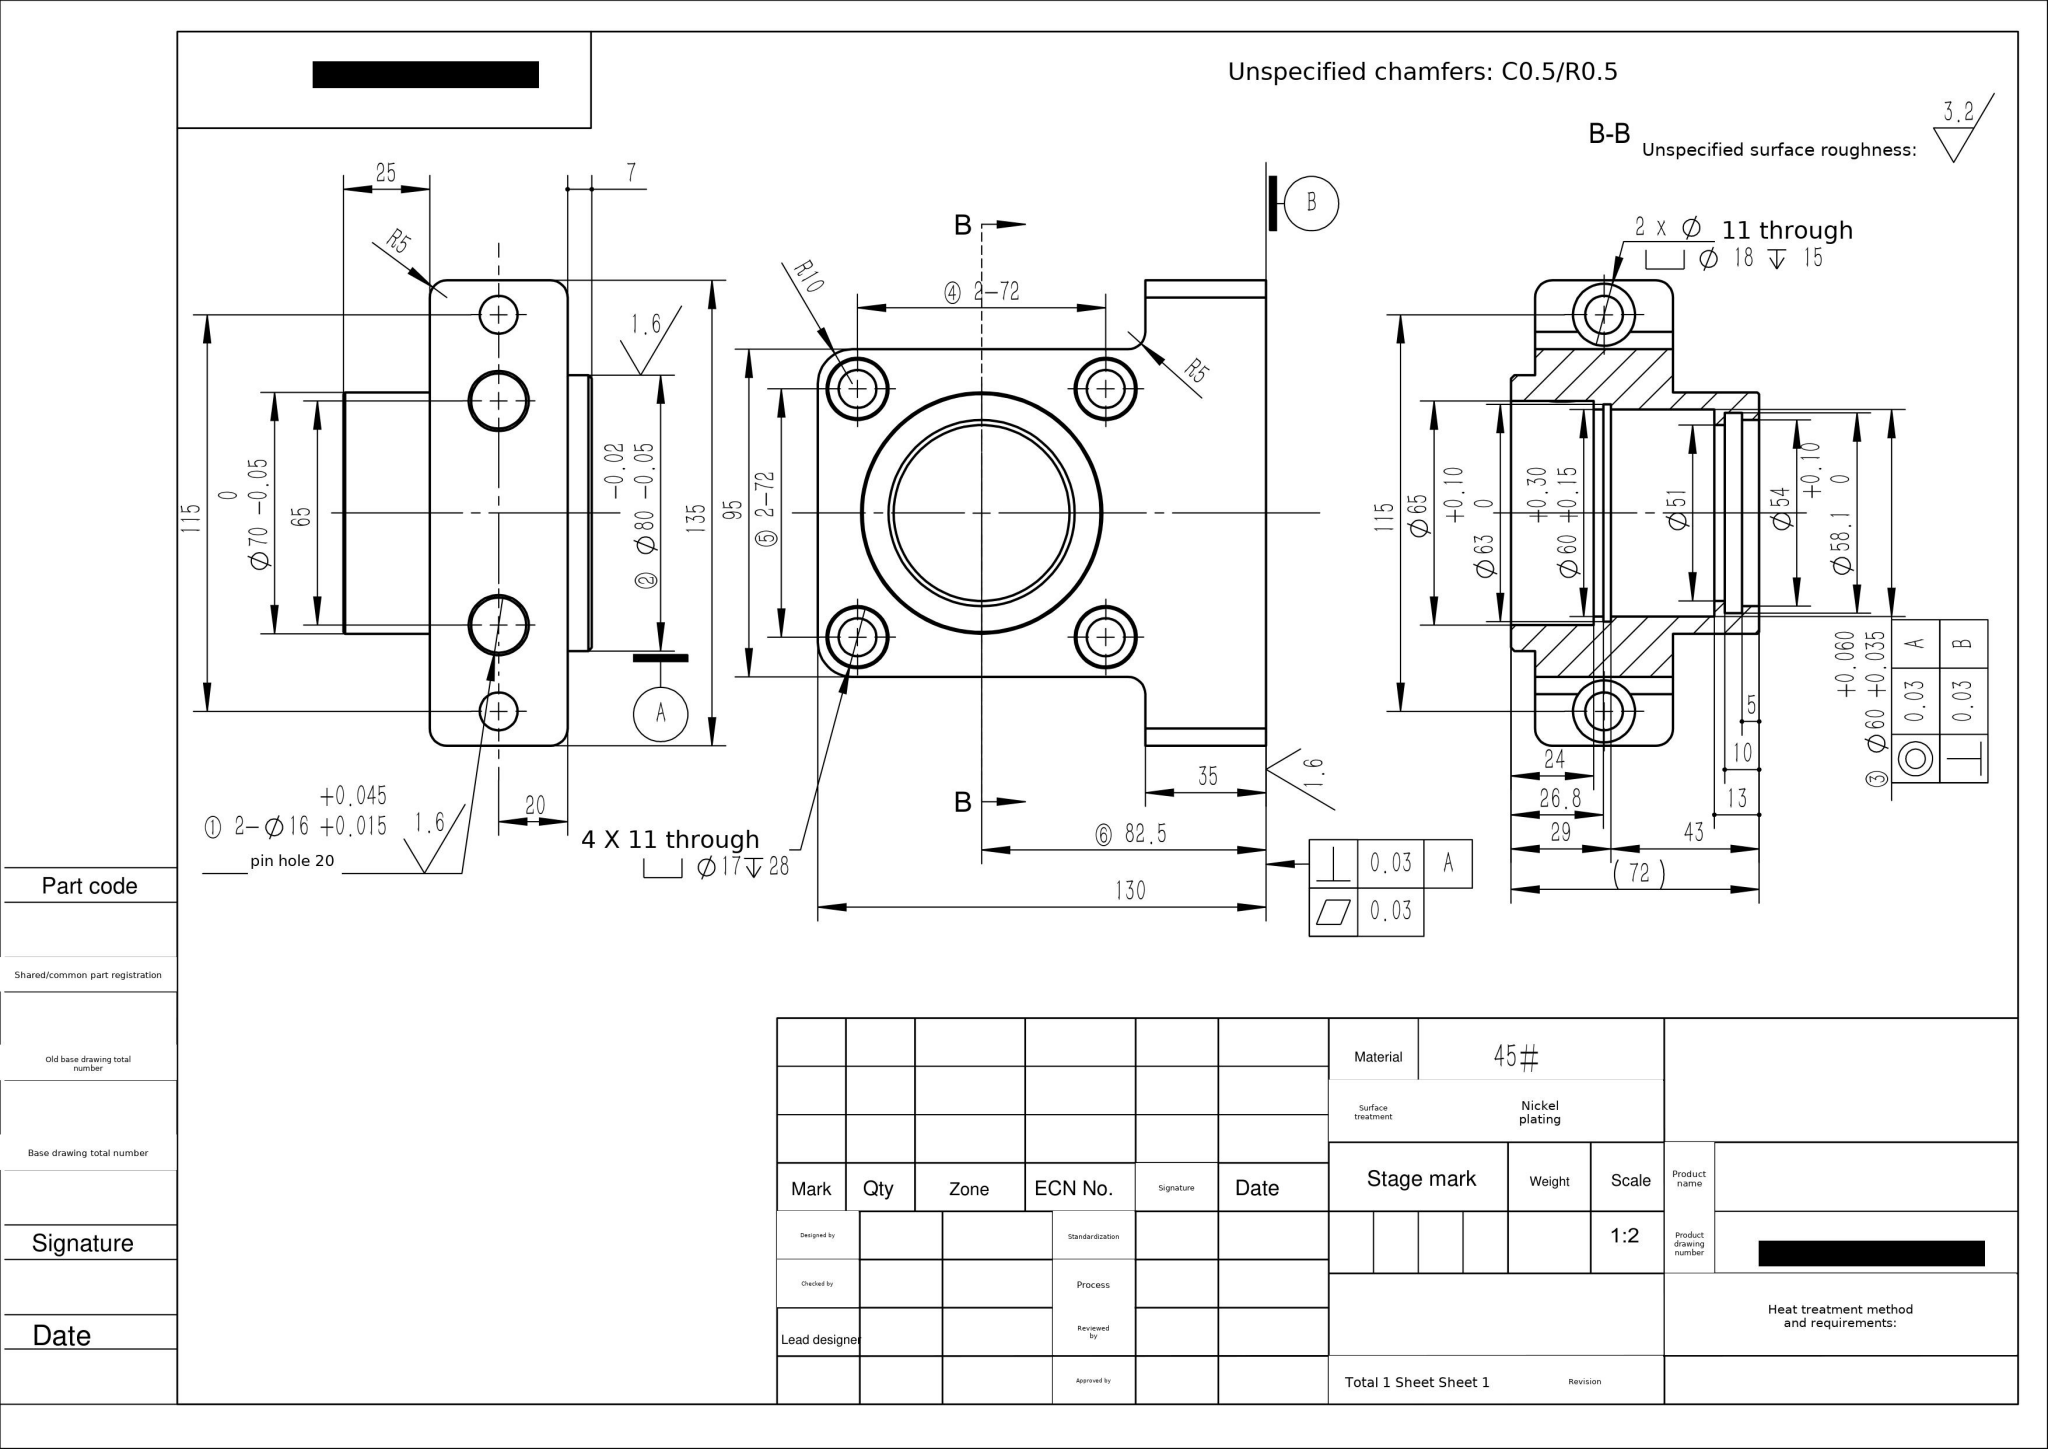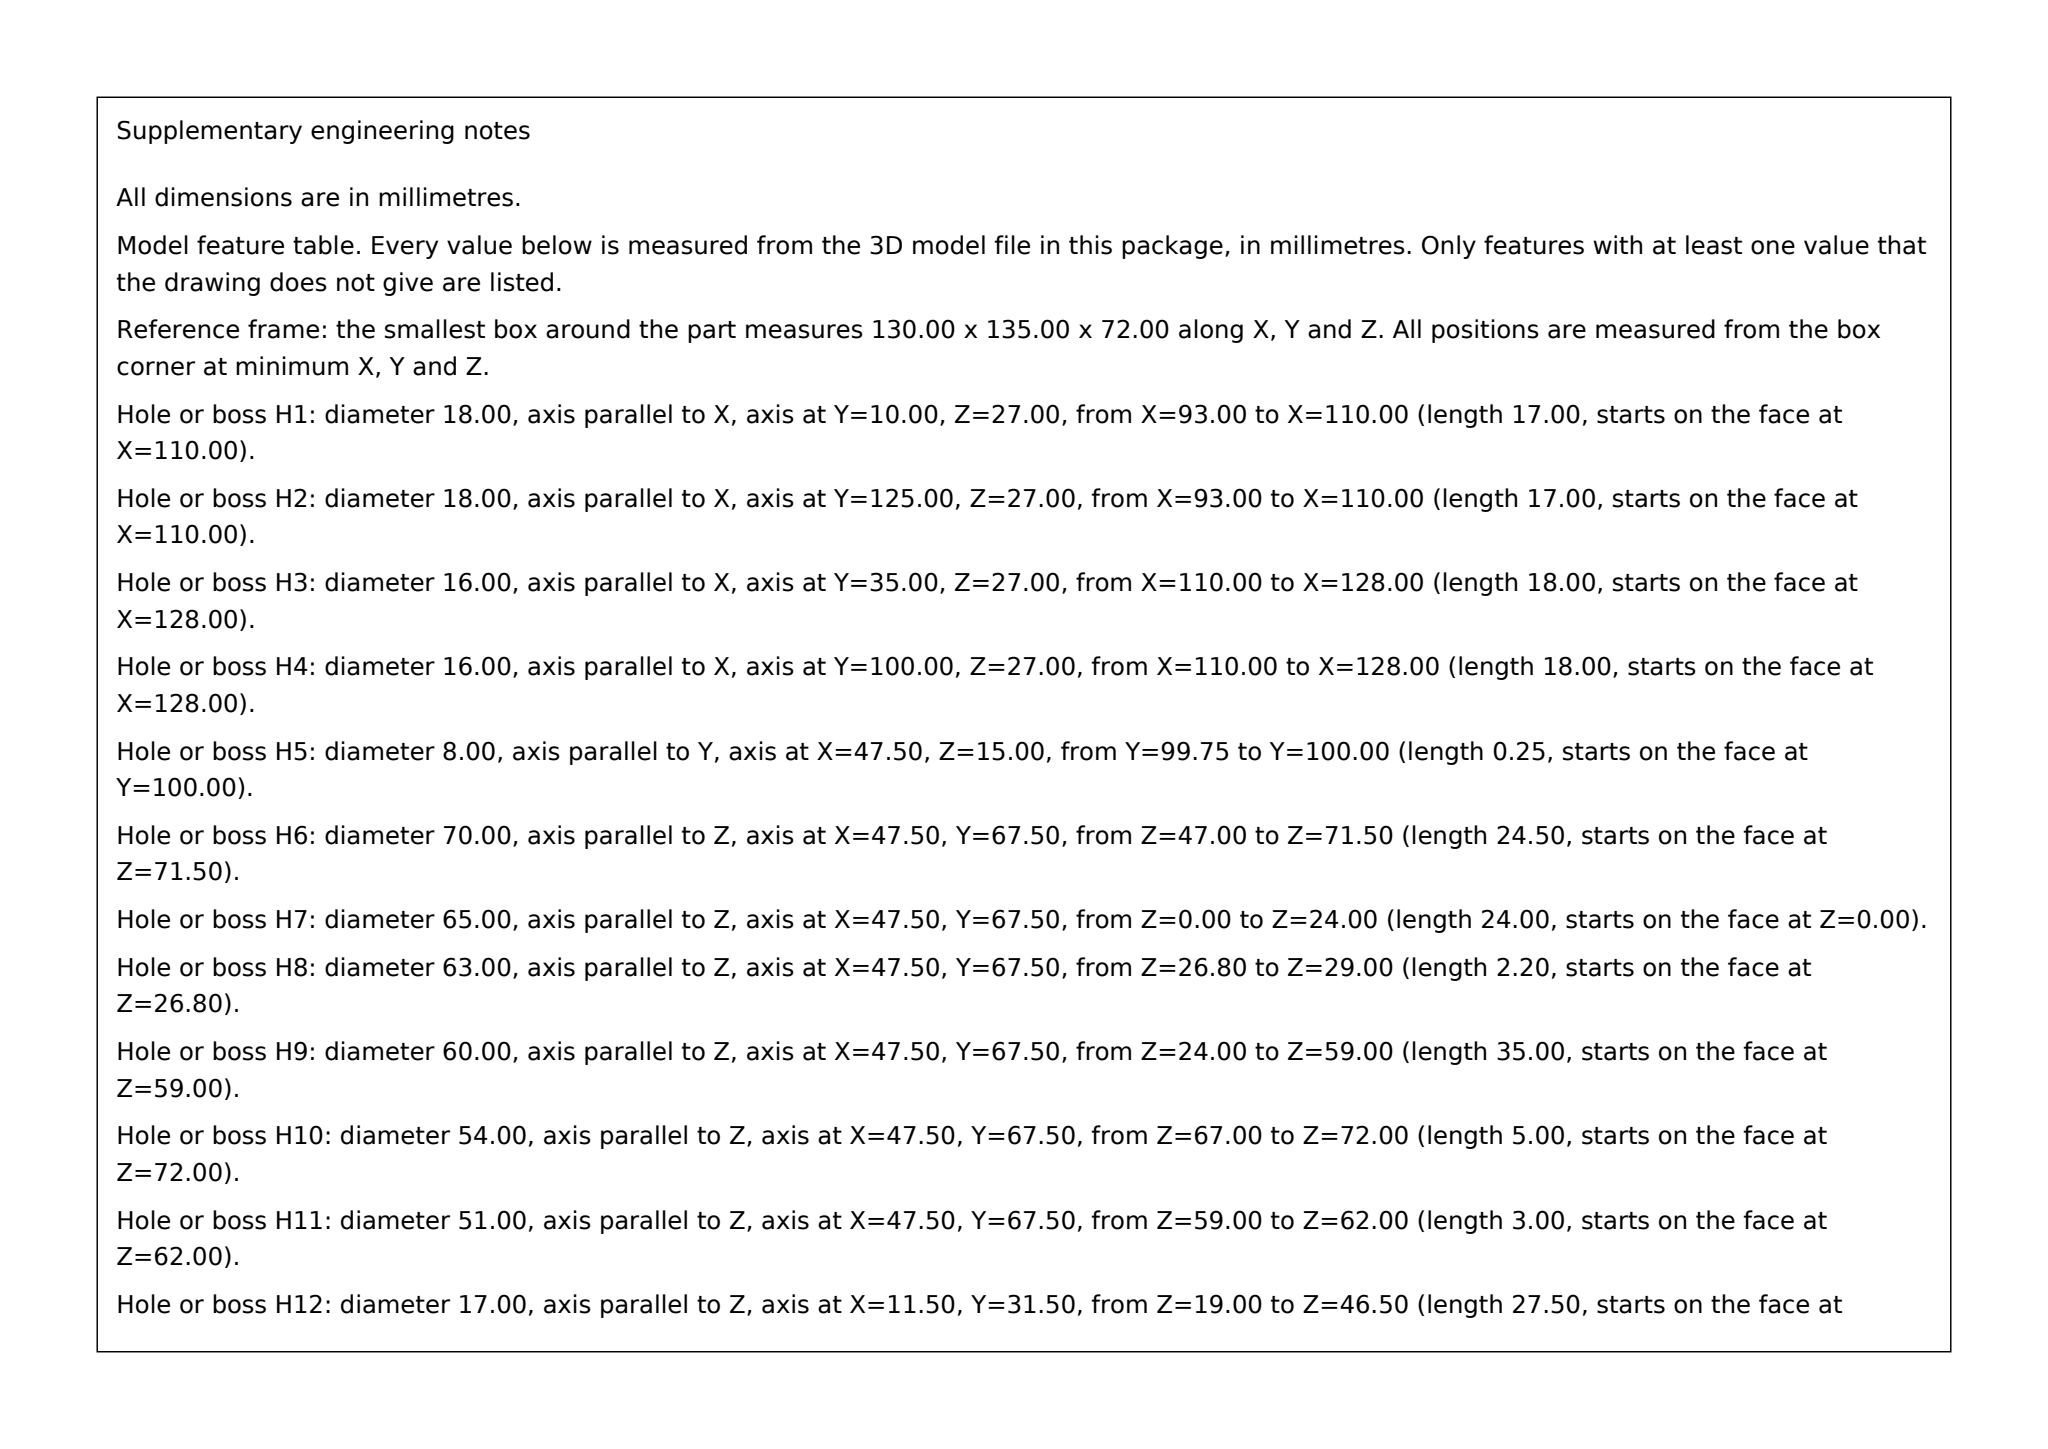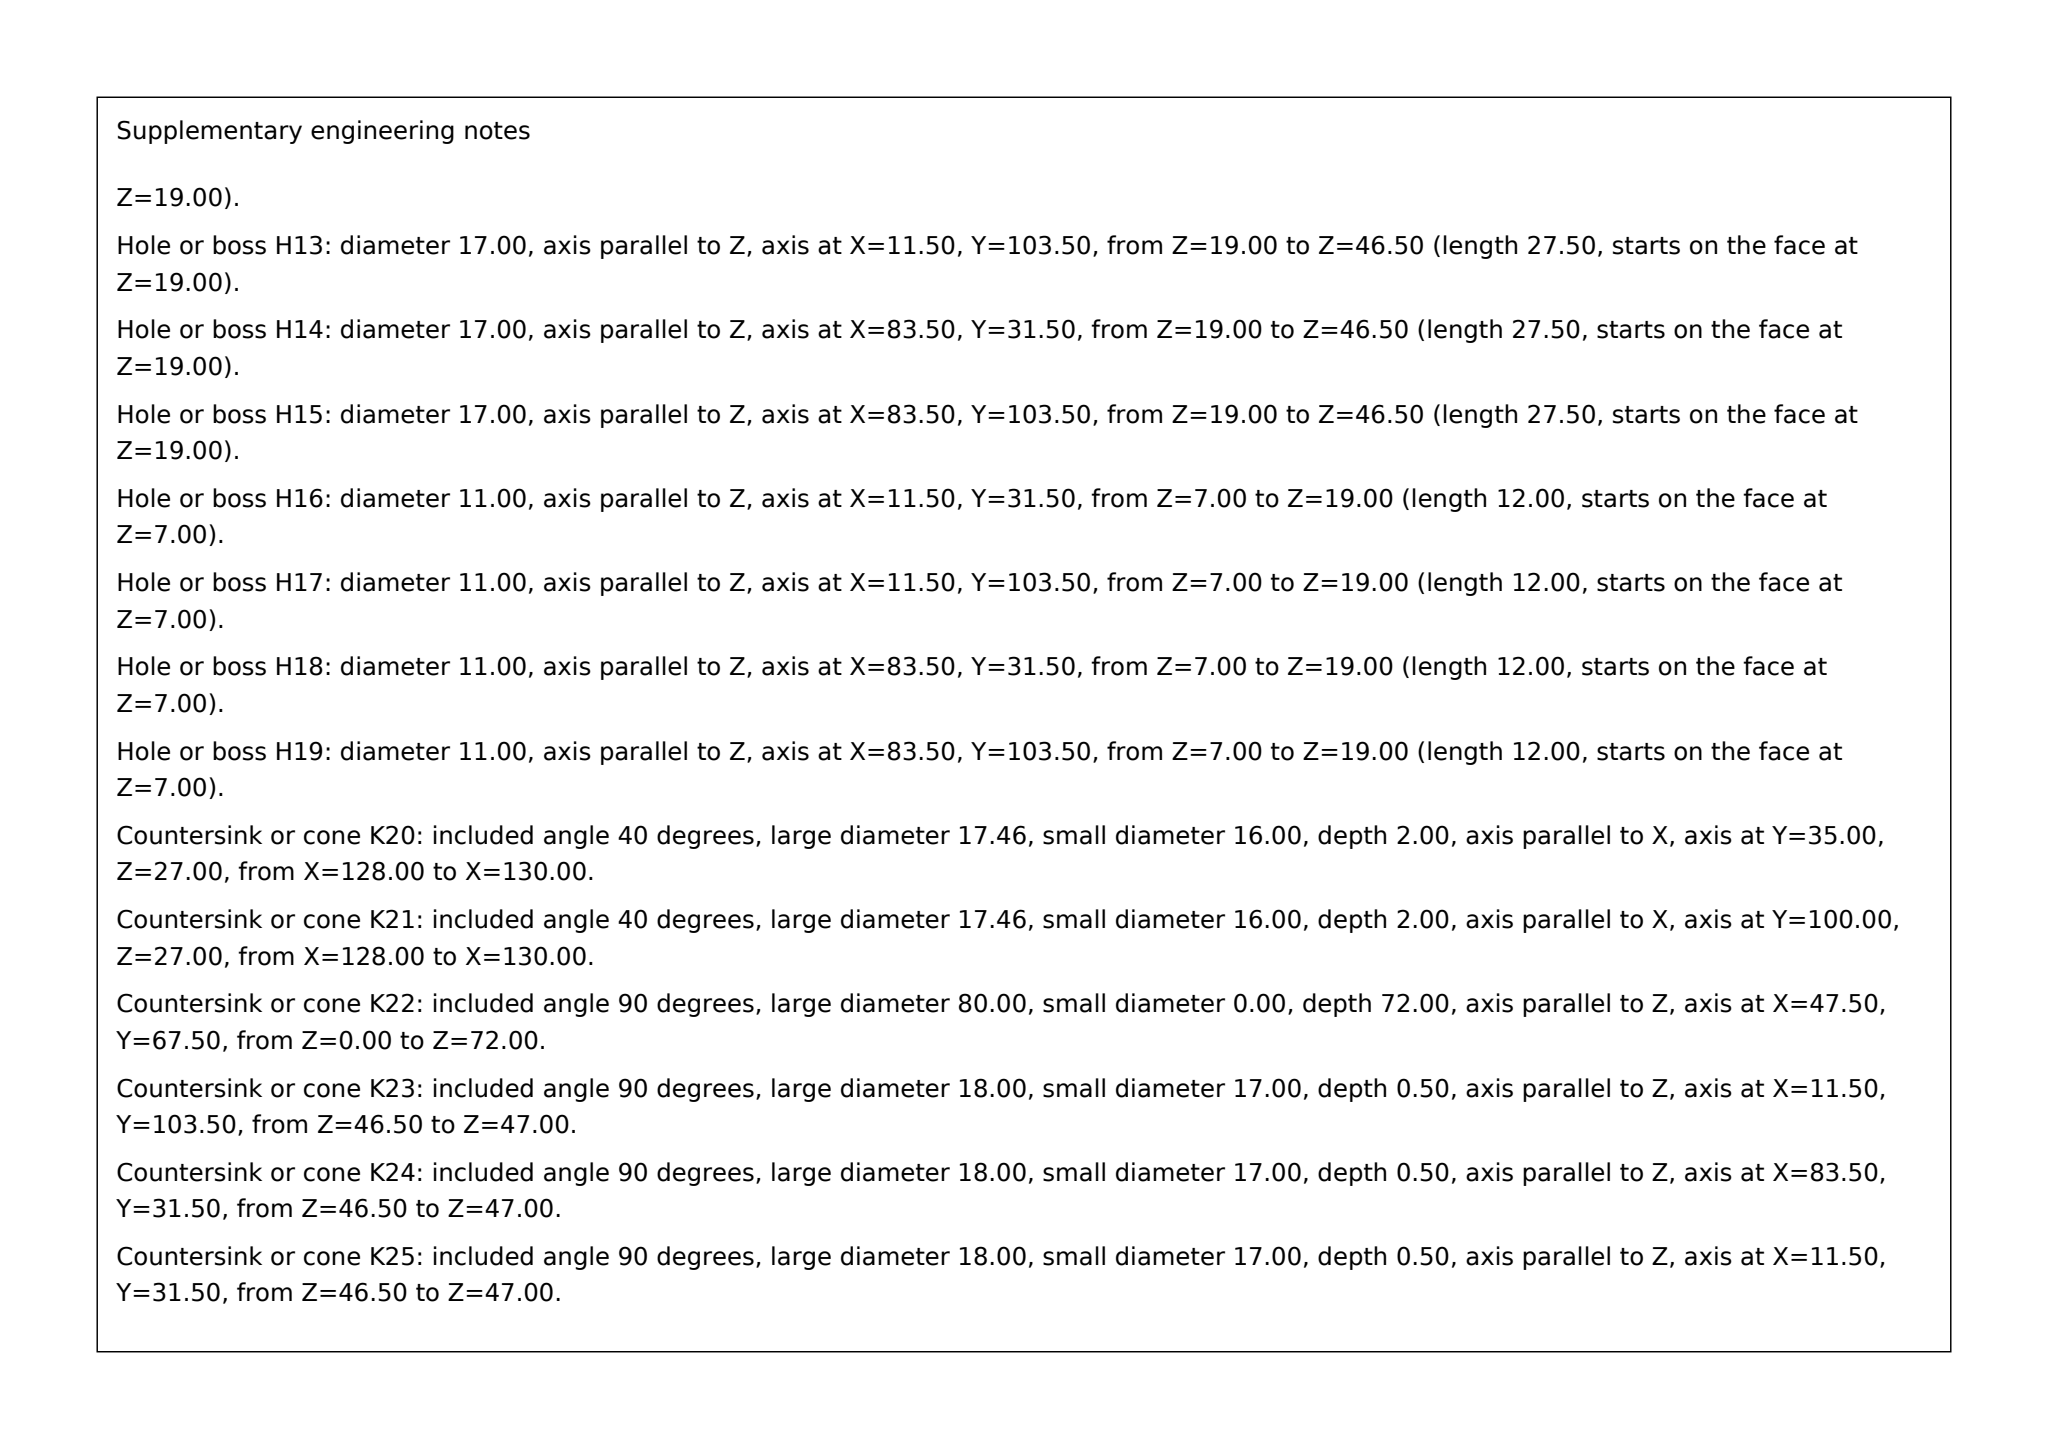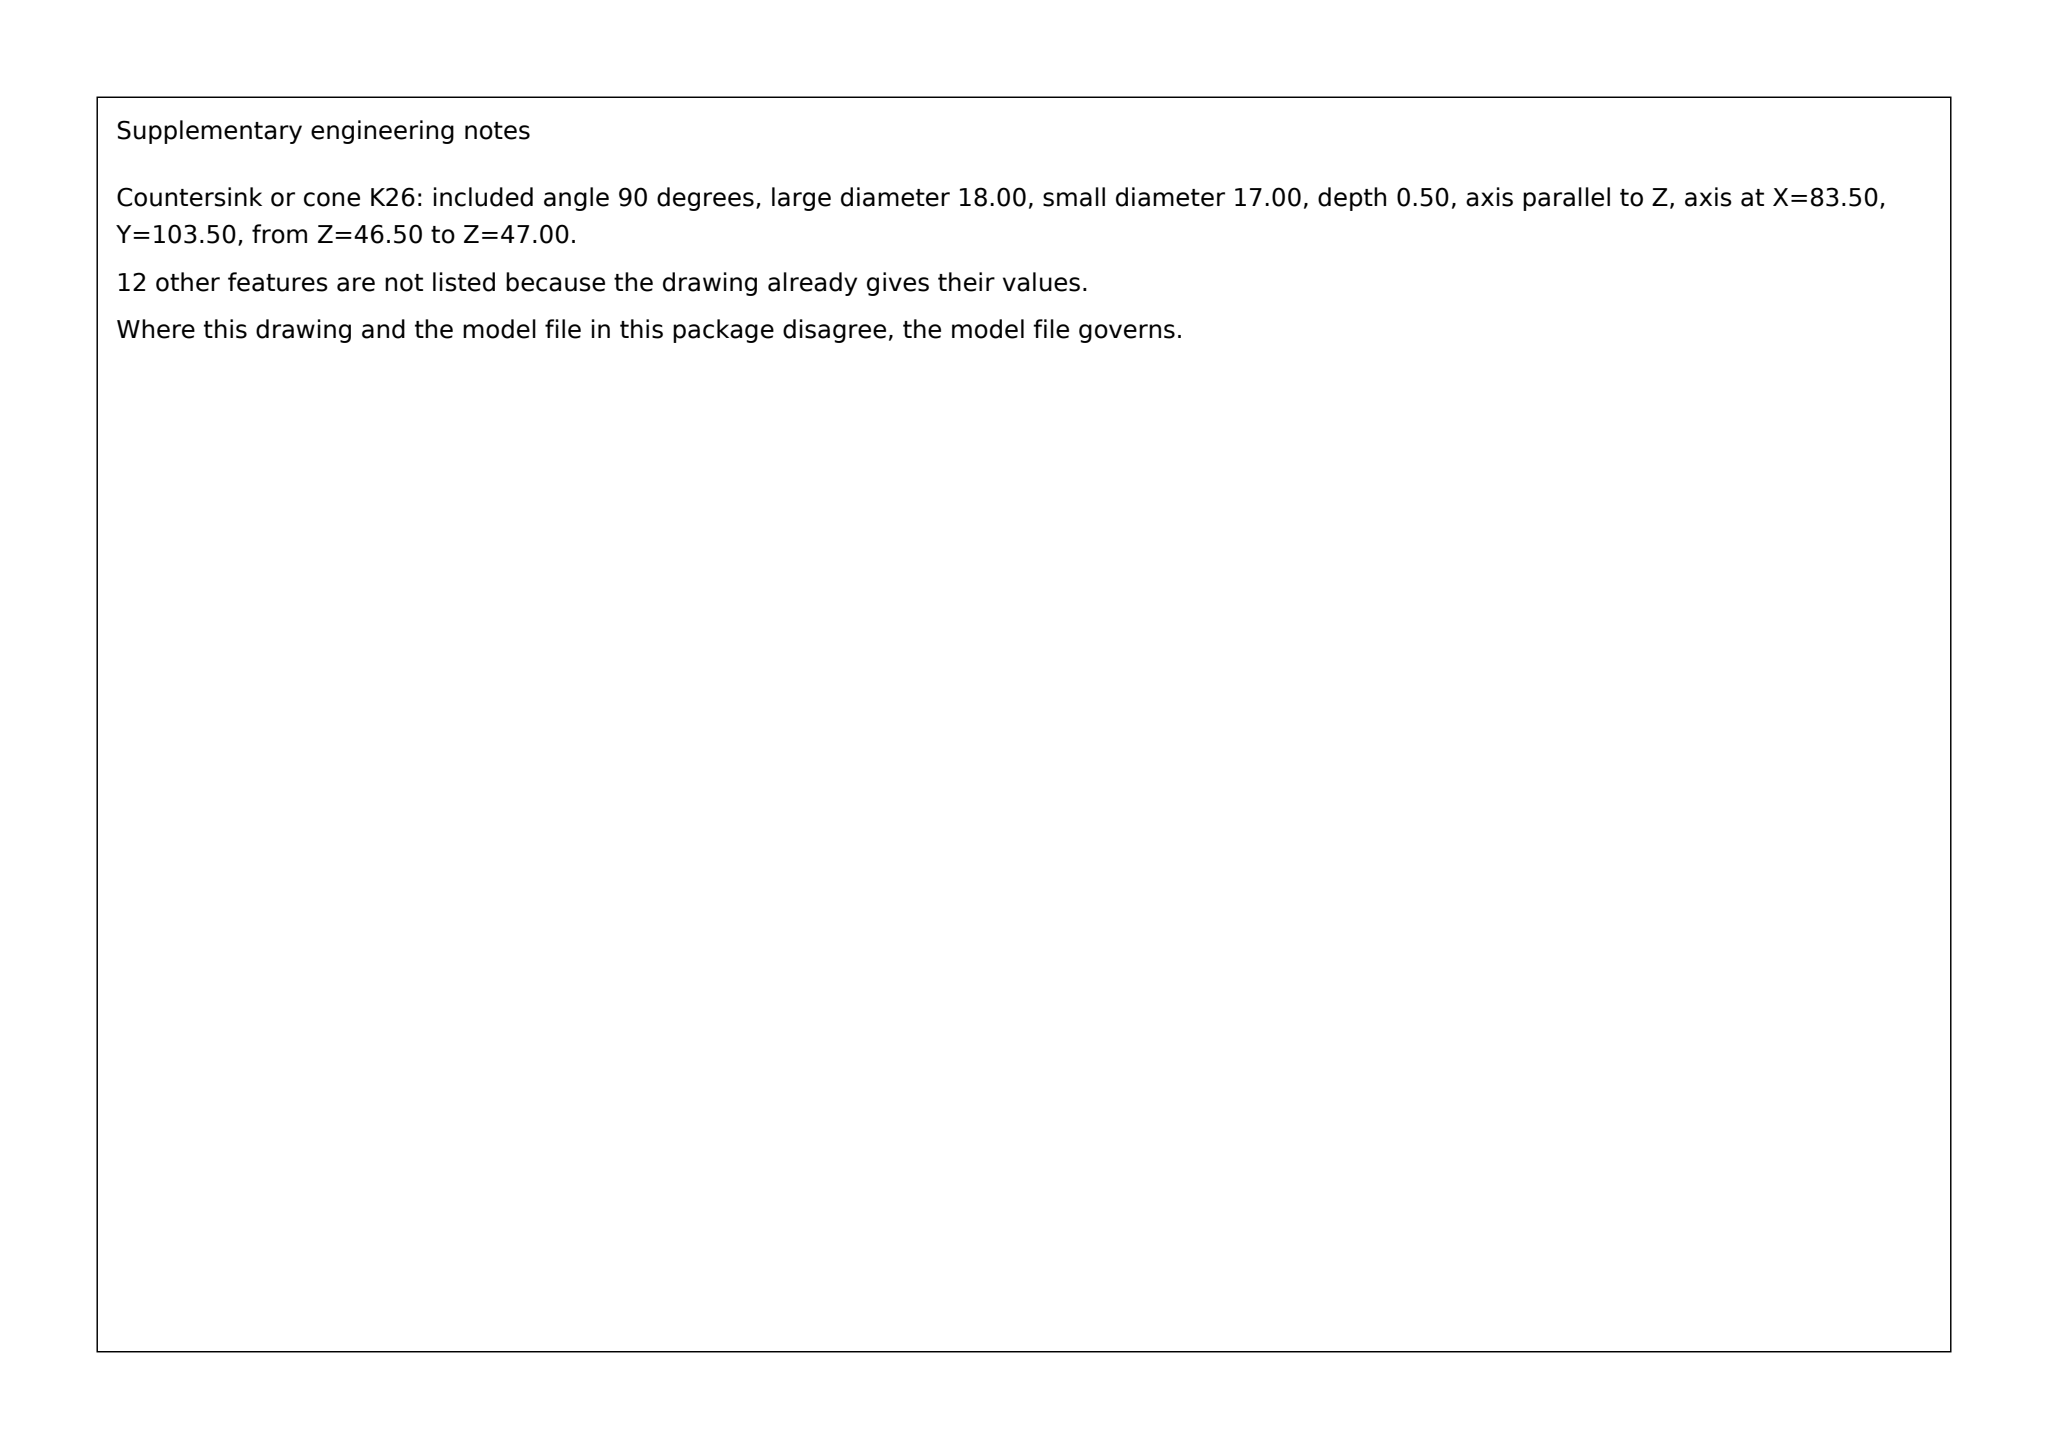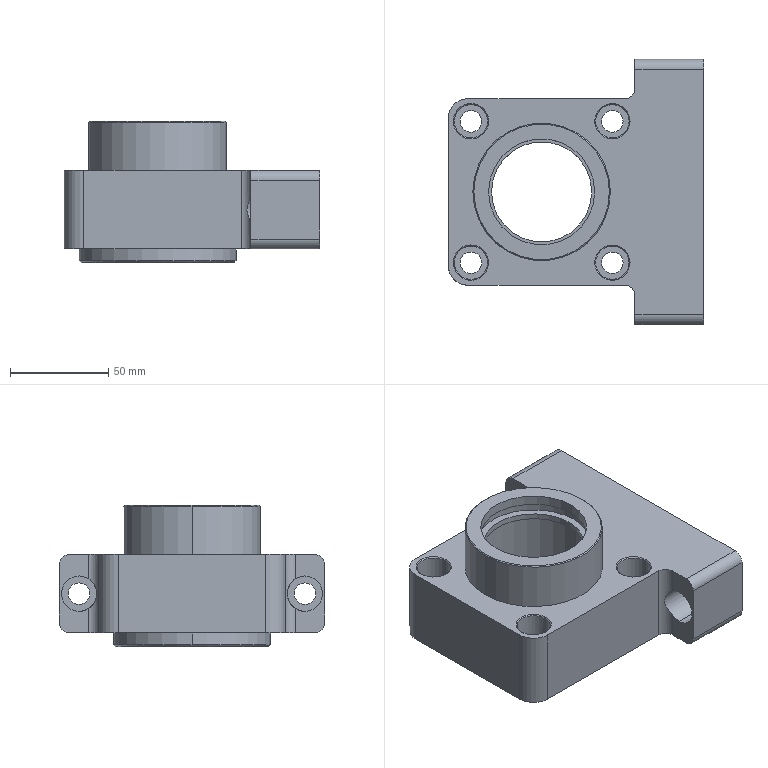Part | SolidWorks | mm | material 45# | 1 solid | 99 faces | box 130 x 135 x 72 mm | volume 419532 mm3 | cylinder 56 | plane 27 | cone 16 | commonest cylinder face diameters 11 x12 17 x8 10 x6 16 x4 18 x4 60 x4 58.1 x2 51 x2